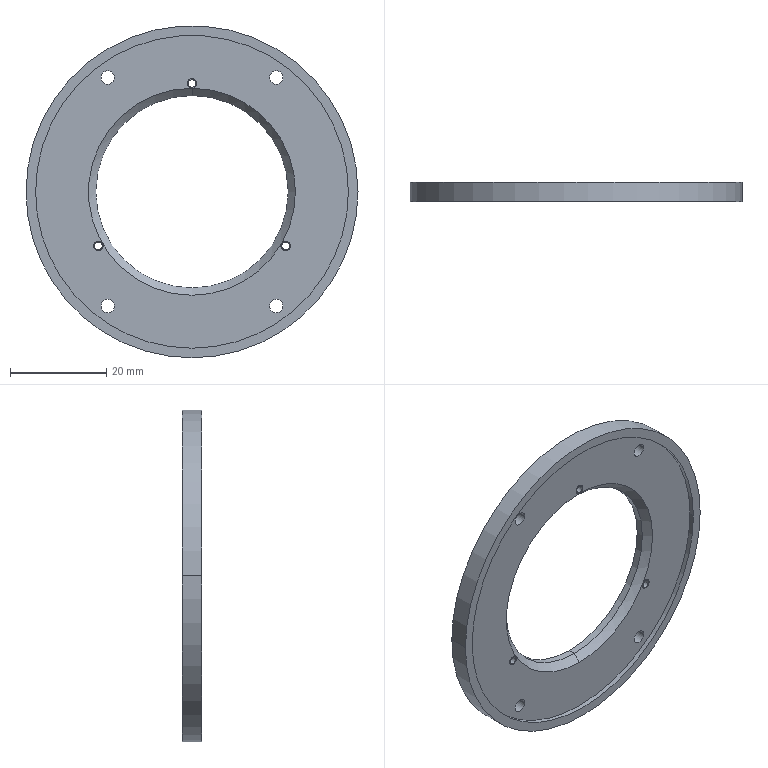CAM job | Mastercam | mm | 1 operations | part box 69 x 4 x 69
1. Drill/Counterbore | 7 - 4 倒角刀